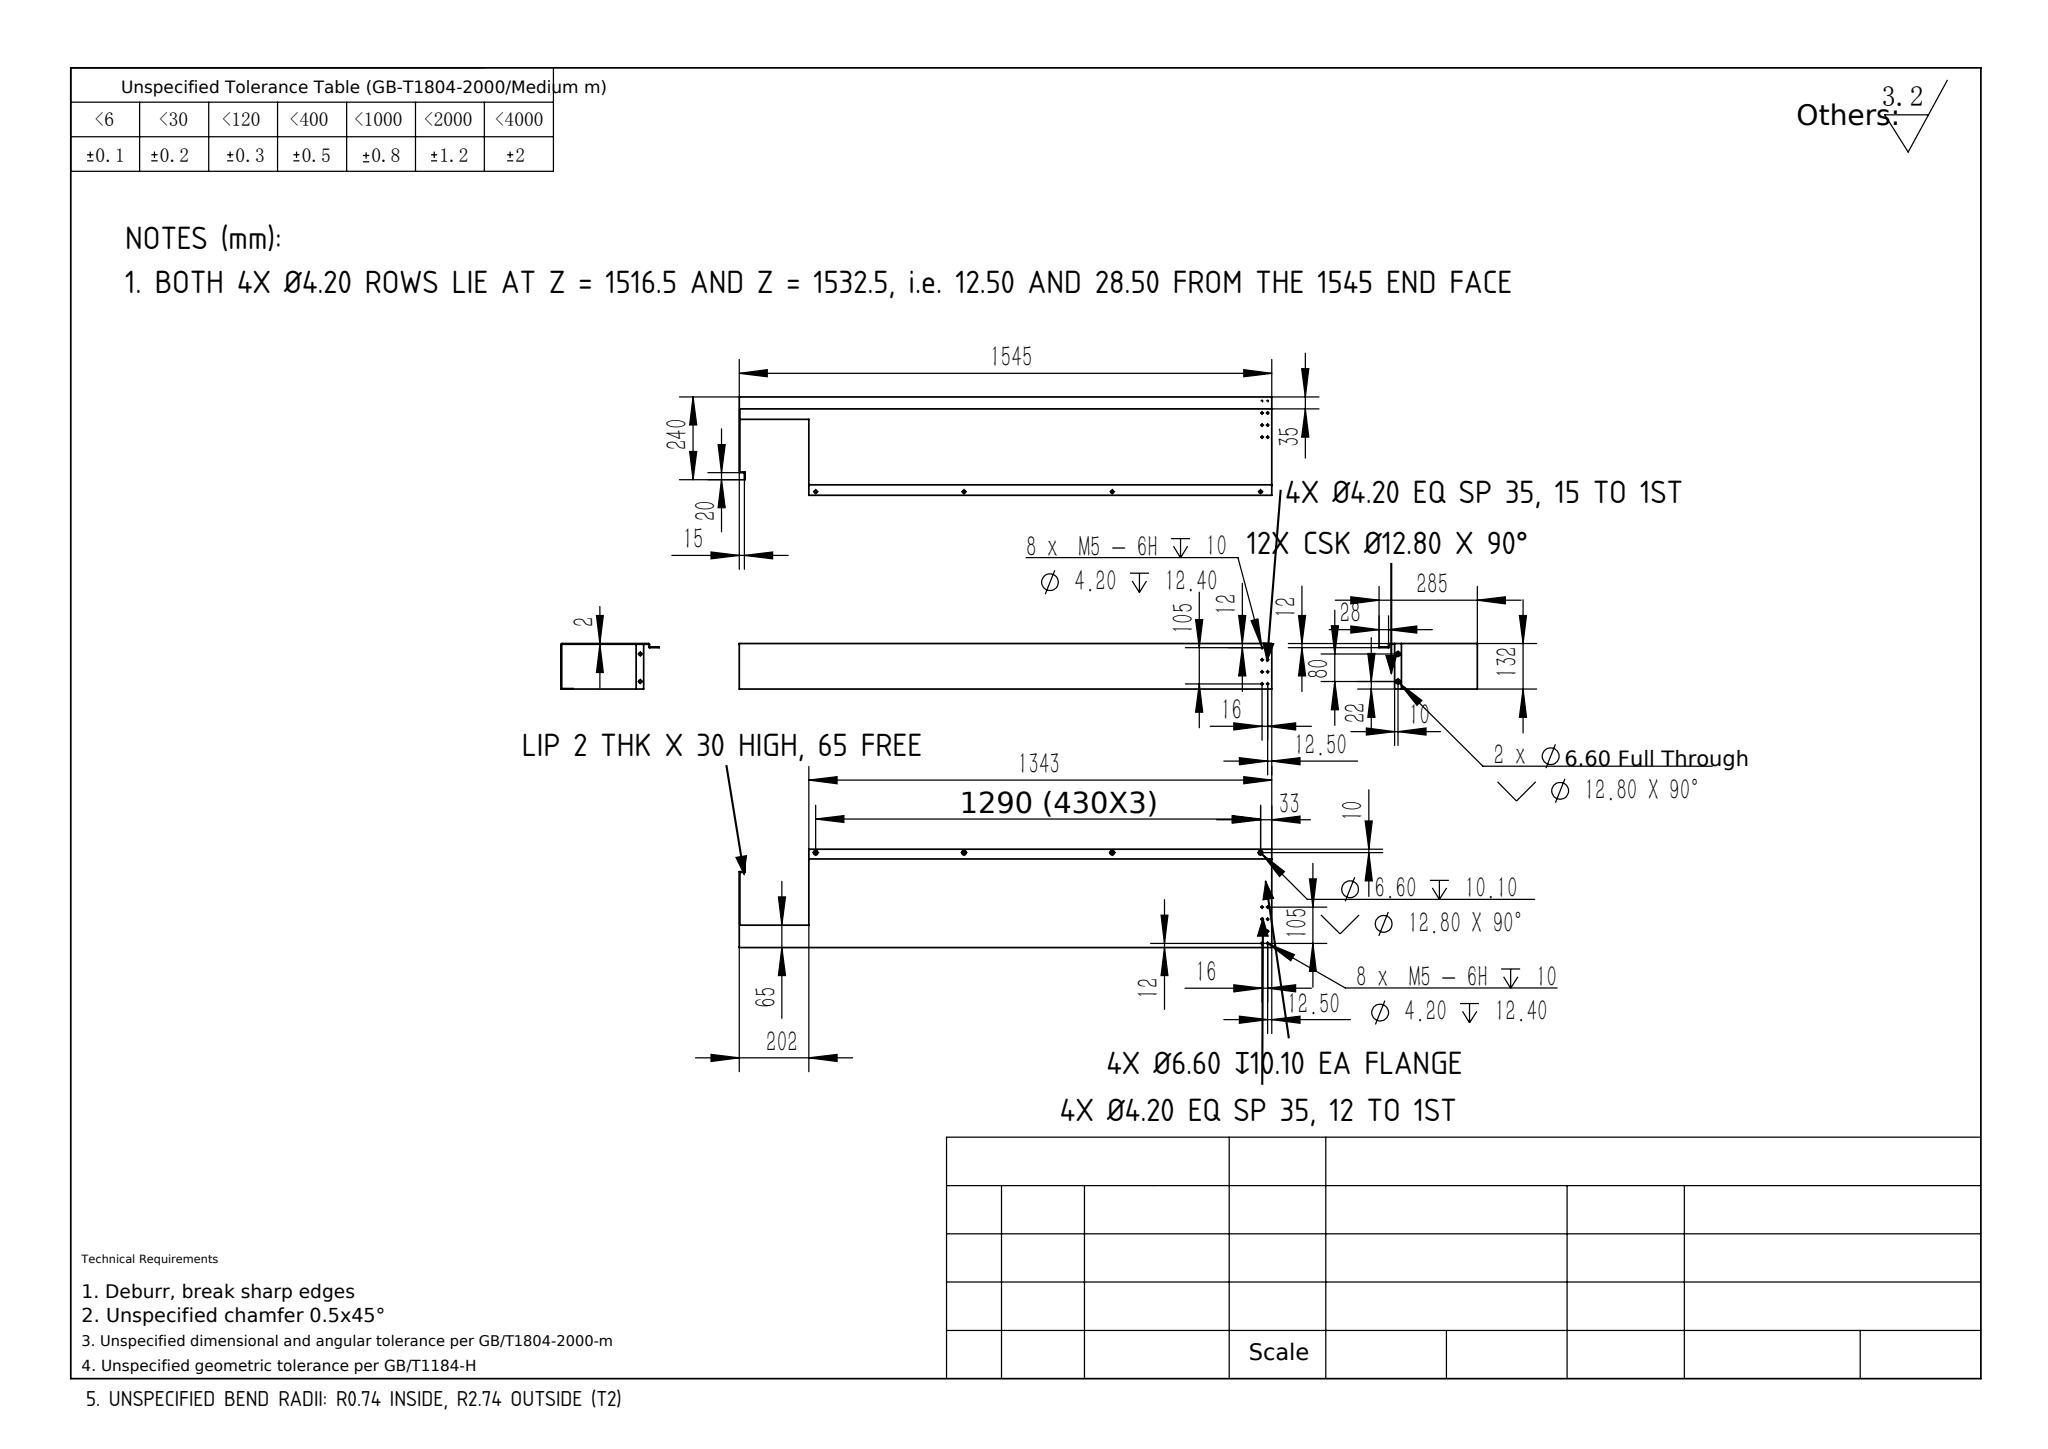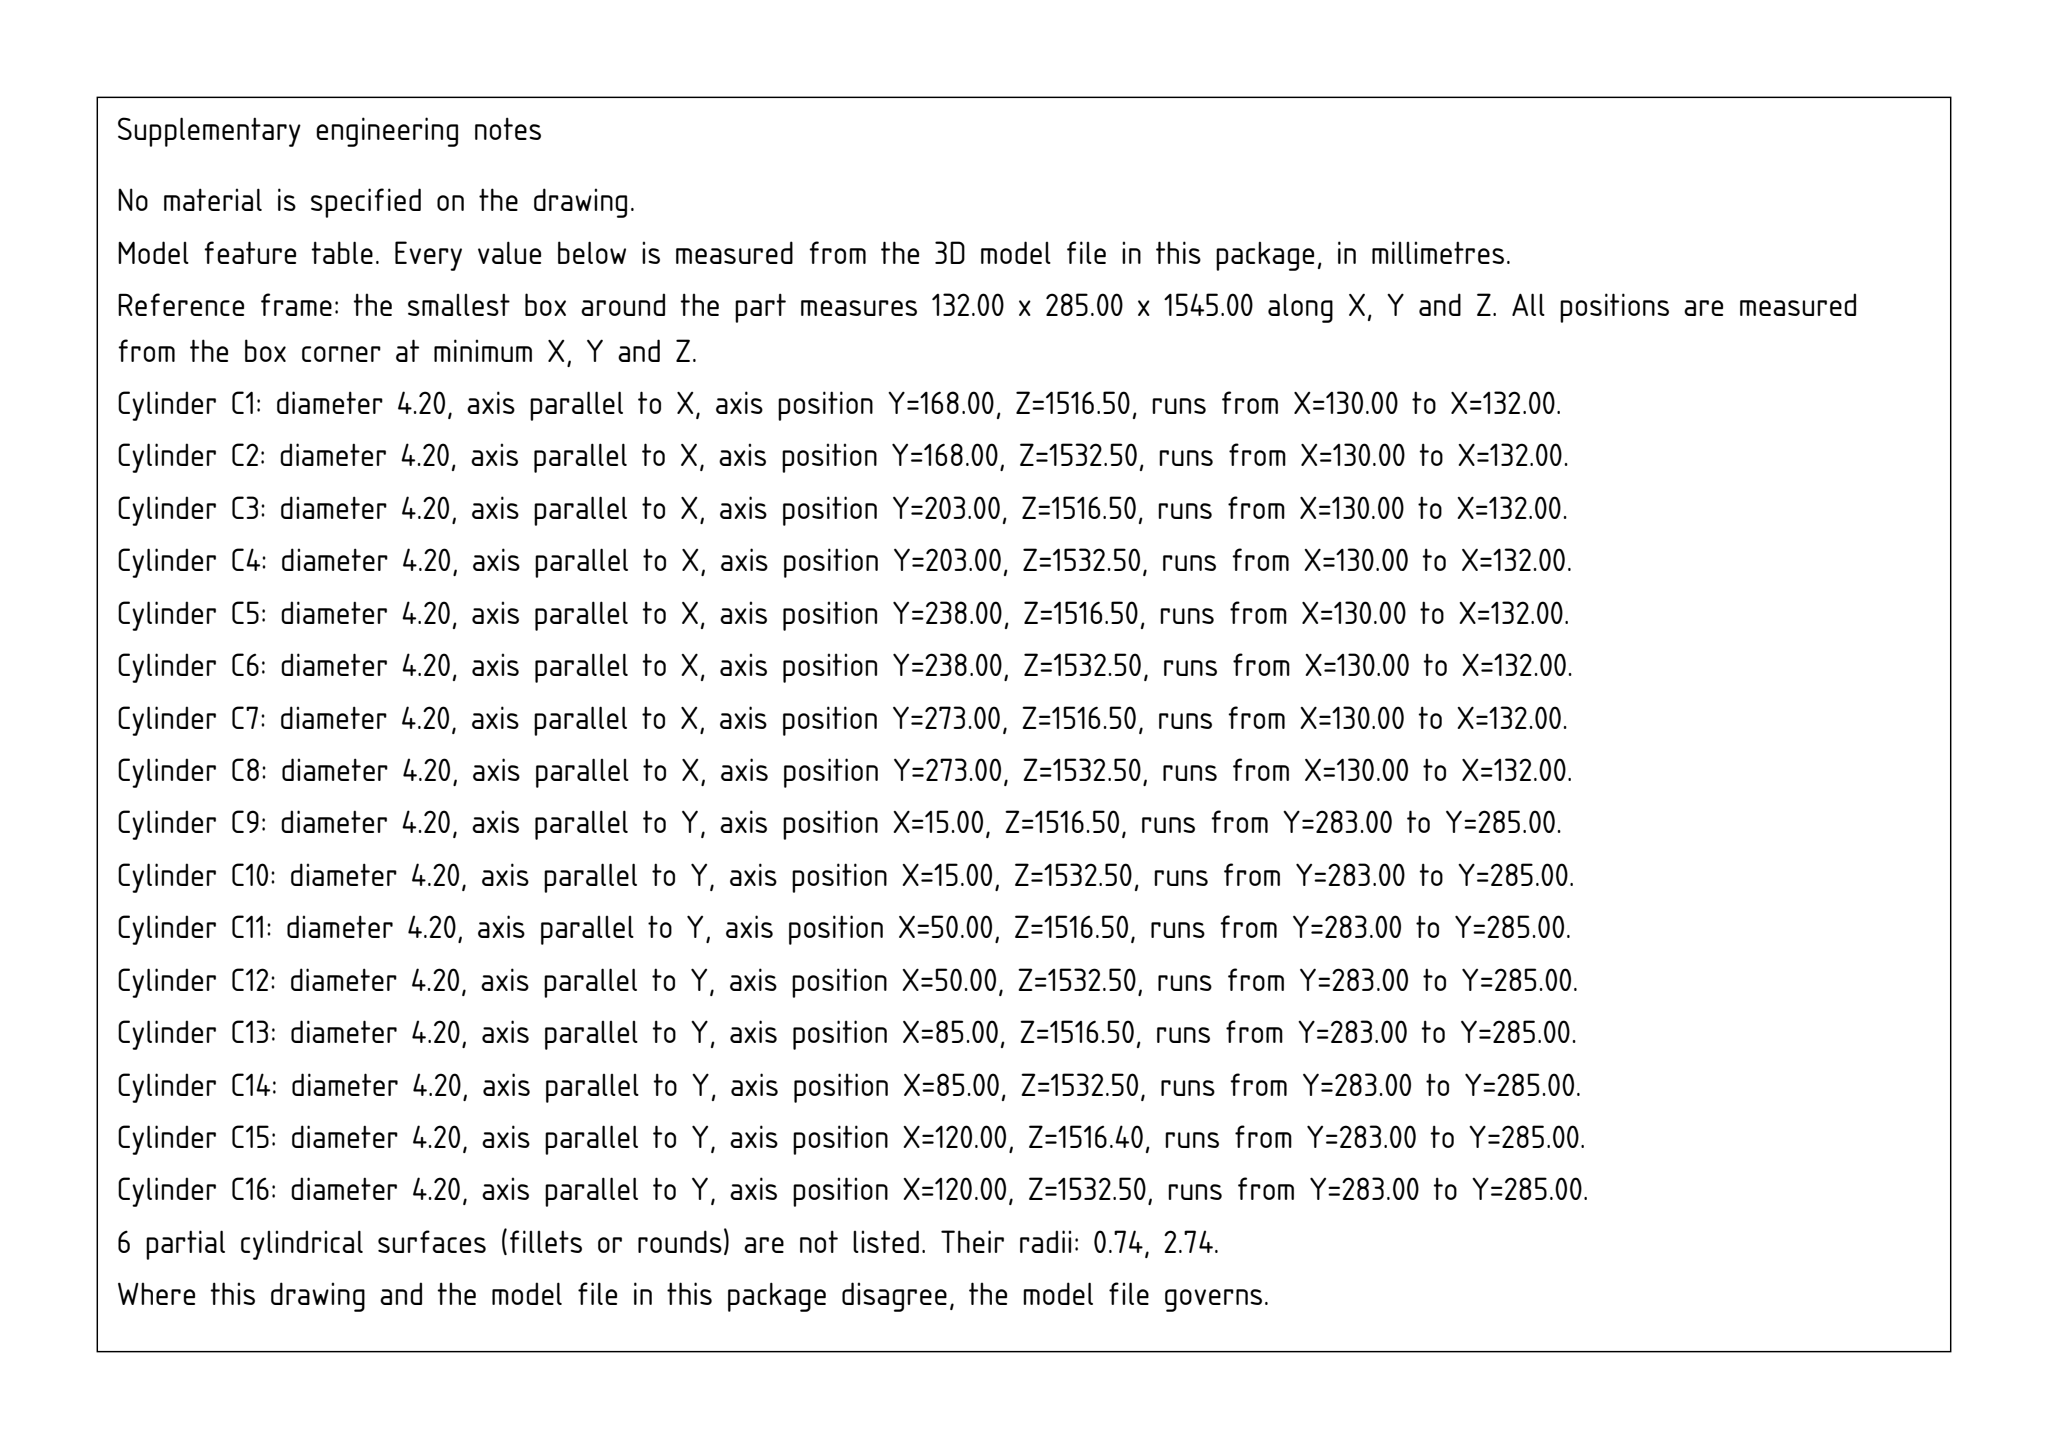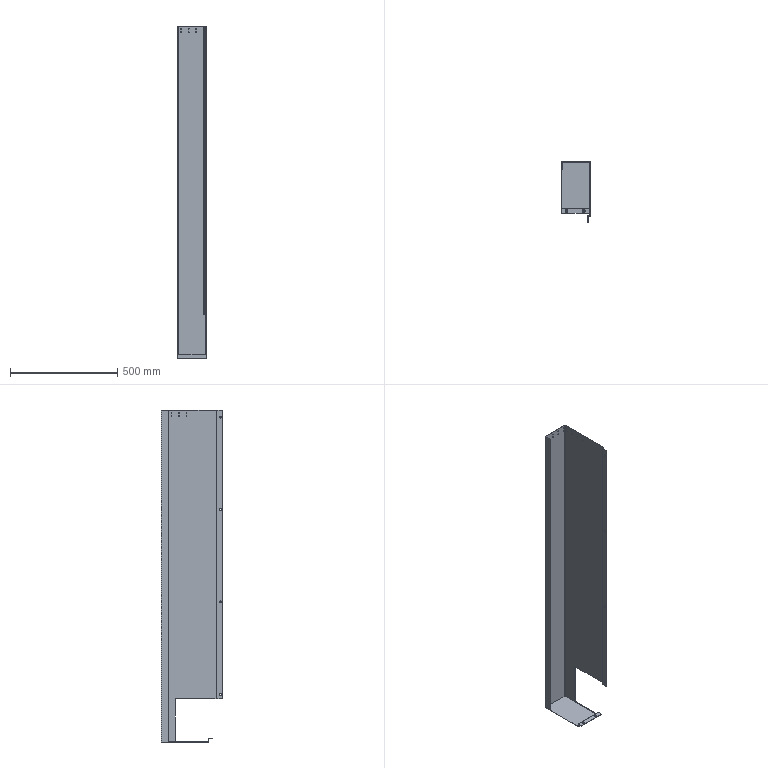Part | SolidWorks | mm | 1 solid | 83 faces | box 132 x 285 x 1545 mm | volume 1380845 mm3 | cylinder 38 | plane 33 | cone 12 | commonest cylinder face diameters 4.2 x32 5.473 x3 1.473 x3
Drawing notes:
UNSPECIFIED BEND RADII: R0.74 INSIDE, R2.74 OUTSIDE (T2) | from the solid: Z-axis bend cylinders dia 1.473 (R0.737 inner) and dia 5.473 (R2.737 outer); wall planes x=0/2, y=283/285 give T2
4 X Ø6.60 DP 10.10, CSK Ø12.80 X 90° EA FLANGE (8 PLACES) | from the solid: cones[90°, ref dia 12.80] count 12 = 8 blind c'sk (4 per flange) + 4 on the 2 X Ø6.60 through holes (c'sk both ends)
CSK Ø12.80 X 90°: 12 PL TOTAL ON PART | from the solid: cones[included_angle,ref_dia]: [90.0, 12.8] occurring 12 times; drawing calls out only 8 + 2 = 10
RETURN LIP 2 THK X 30 HIGH; FREE EDGE 65 FROM 285 O/A FACE | from the solid: axis_planes x=120.0 & x=122.0 (2 thk lip); y=220.0 & y=250.0 faces -> 30 high; 285.0-220.0=65 from the y=285 outer face used by the 285 o/a dim
4X Ø4.20 (M5-6H) HOLES EQ SP ON 35 PITCH (3 X 35 = 105 O/A); FIRST HOLE 15 FROM THE X=0 SIDE FACE OF THE 132 WIDE FLANGE | from the solid: cylinders dia 4.20 axis y at x = 15.0, 50.0, 85.0, 120.0 (uniform 35 pitch, 105 span)
4X Ø4.20 (M5-6H) HOLES EQ SP ON 35 PITCH (3 X 35 = 105 O/A); FIRST HOLE 12 FROM THE 285 O/A FACE (Y=285) | from the solid: cylinders dia 4.20 axis x at y = 168.0, 203.0, 238.0, 273.0 (285 - 273 = 12, uniform 35 pitch)
BOTH 4X Ø4.20 ROWS LIE AT Z = 1516.5 AND Z = 1532.5, i.e. 12.50 AND 28.50 FROM THE 1545 END FACE | from the solid: cylinders dia 4.20 at z = 1516.5 and 1532.5; axis_planes z = 1545.0 (end face)